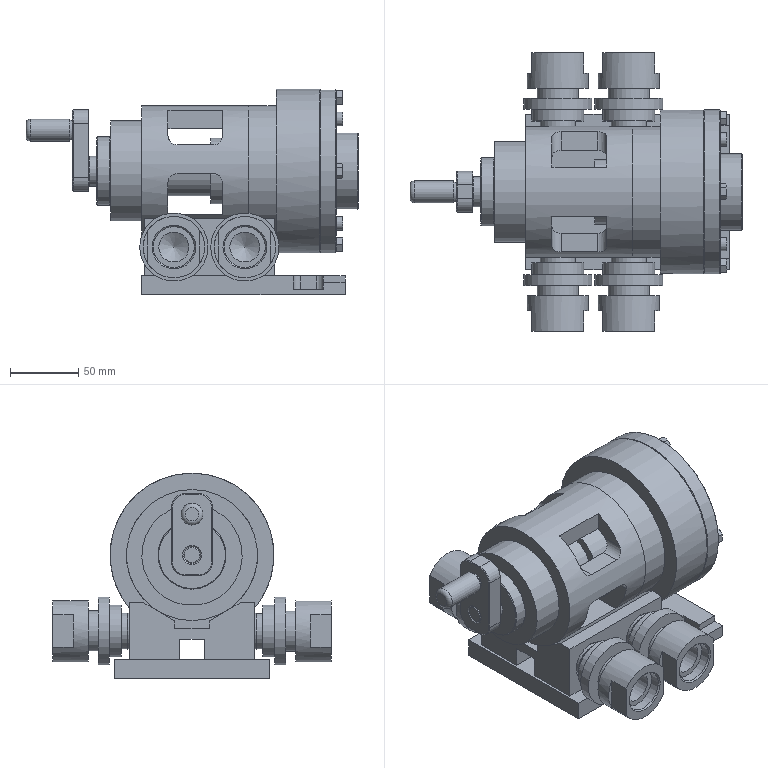Assembly | NX | mm | 24 component files | 24 solids | 507 faces | box 243.2 x 204 x 150.64 mm | volume 1705210 mm3 | plane 244 | cylinder 171 | cone 91 | torus 1 | commonest cylinder face diameters 4 x24 10 x15 5 x12 6 x10 30 x9 26.59 x8 13.6 x8 8.5 x6
Bill of materials:
unnamed part 1 | 4 |  | Hex-head bolt-like part: hexagonal head with chamfered outer corners and a round bearing face, joined to a plain cylindrical shank with a chamfered tip.
unnamed part 2 | 1 |  | Impeller-like disc: a flat circular back plate with several curved, spiral-shaped vanes standing up from one face, and a central round bore with a single keyway notch.
unnamed part 3 | 2 |  | Socket-head cap-screw-like part: a cylindrical head with a recessed drive socket in its end face, on a plain cylindrical shank with a chamfered tip.
unnamed part 4 | 4 |  | Stepped turned body of revolution: a large cylindrical section with an end bore and one flat machined on its side, a raised collar, several smaller stepped diameters, and a small chamfered spigot at the far end.
unnamed part 5 | 1 |  | Stepped casing-like body with three coaxial diameters. The large end face carries six small hole features on a circle, and the end has an internal cavity with a curved, off-center wall and a tongue-like edge, plus a central round opening.
unnamed part 6 | 1 |  | Stepped cylindrical pin: a long main body with a rounded/filleted outer end, a chamfered step down to a reduced neck, a groove, and a short end section with a chamfered tip.
unnamed part 7 | 1 |  | Flanged hub: a thin circular flange with six through holes evenly spaced on a bolt circle, a raised cylindrical hub on one face, and a central through bore.
unnamed part 8 | 1 |  | Rounded-rectangle plate (spacer/link-like) with two identical round through holes along its long axis.
unnamed part 9 | 2 |  | Plain solid cylinder with small chamfers on both end edges (dowel/pin-like).
unnamed part 10 | 1 |  | Cylindrical housing/cage: a large thin-walled cylinder with rounded-rectangular windows cut through opposite sides, a smaller-diameter spigot step at one end, an open large bore at the other end, and six small holes in that end face.
unnamed part 11 | 1 |  | Plain solid prism with an obround (stadium-shaped) cross-section: flat parallel sides joined by semicircular ends, extruded to a constant length.
unnamed part 12 | 1 |  | Rectangular V-block-like part: the top has two sloped faces forming a V-shaped trough with a central rectangular slot, the underside has a rectangular through channel along its length, and one face has two round holes with conical (drill-point) bottoms.
unnamed part 13 | 1 |  | Stepped rotationally symmetric shaft. From one end: a short small-diameter end stub, a short collar, a large thin flange, a long main cylindrical body, a long reduced-diameter section, and a short small-diameter end journal. There is an elongated slot-like recess on the reduced section near the journal end.
unnamed part 14 | 2 |  | Solid two-step cylindrical pin or stud: a short large-diameter base cylinder with a smaller coaxial cylinder rising from it. Both the free end of the small cylinder and the outer bottom edge of the base are chamfered.
unnamed part 15 | 1 |  | Flat rectangular plate with four small round through holes in a scattered pattern and one larger round through hole near one end. One edge has cutouts: an open slot with a rounded inner end, a second slot-like cutout, and small stepped notches along the edge profile.
Mates:
1. fix | base_plate 1 component
2. concentric | bracket 1 edge | base_plate 1 edge
3. parallel | bracket 1 face | base_plate 1 face
4. center | bracket 1 face | bracket 1 face | bushing 1 face
5. touch align | bushing 1 face | base_plate 1 face
6. touch align | bushing 1 face | bracket 1 face
7. concentric | volute_casing 1 arc | bushing 1 edge
8. touch align | volute_casing 1 face | bushing 1 face
9. concentric | volute_casing 1 edge | end_cap 1 edge
10. distance | volute_casing 1 face | end_cap 1 face
11. concentric | bushing 1 edge | spindle 1 edge
12. concentric | rocker 1 edge | swivel_plate 1 edge
13. parallel | impeller 1 face | spindle 1 face
14. concentric | impeller 1 edge | volute_casing 1 edge
15. parallel | bushing 1 face | bracket 1 face
16. bond | swivel_plate 1 component | spindle 1 component
17. concentric | bracket 1 edge | pivot_shaft 4 edge
18. parallel | pivot_shaft 4 face | bracket 1 face
19. concentric | bracket 1 edge | pivot_shaft 3 edge
20. parallel | pivot_shaft 3 face | bracket 1 face
21. concentric | bracket 1 edge | pivot_shaft 2 edge
22. parallel | pivot_shaft 2 face | base_plate 1 face
23. concentric | bracket 1 edge | pivot_shaft 1 edge
24. parallel | pivot_shaft 1 face | base_plate 1 face
25. concentric | bracket 1 edge | pin 2 edge
26. concentric | bracket 1 edge | pin 1 edge
27. concentric | screw_m8_5 2 edge | base_plate 1 edge
28. concentric | screw_m8_5 1 edge | base_plate 1 edge
29. concentric | bolt 2 edge | end_cap 1 edge
30. concentric | bolt 1 edge | end_cap 1 edge
31. concentric | end_cap 1 edge | screw_m5x20 4 edge
32. fix | assembly component
33. bond | screw_m5x20 4 component | assembly component
34. bond | screw_m5x20 3 component | assembly component
35. bond | screw_m5x20 2 component | assembly component
36. bond | screw_m5x20 1 component | assembly component
37. circular | assembly datumaxis | assembly cartesiancoordinatesystem | assembly cartesiancoordinatesystem | assembly cartesiancoordinatesystem | assembly cartesiancoordinatesystem
38. concentric | key 1 arc | spindle 1 edge
39. parallel | key 1 face | spindle 1 face